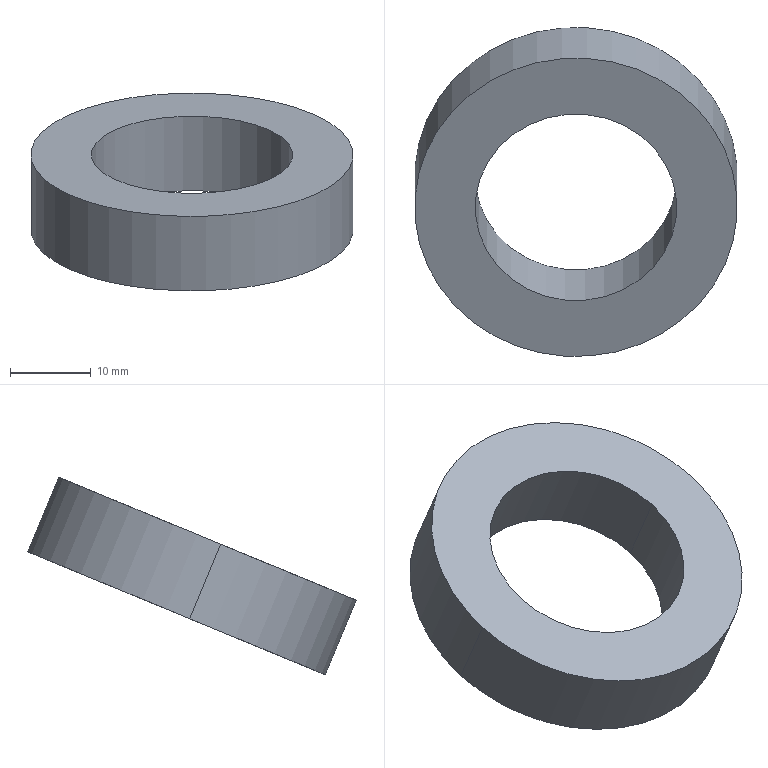Component | SolidWorks | FixedBushing-2 | 1 solid | 6 faces | box 40 x 40.79 x 24.52 mm | volume 7658 mm3 | cylinder 4 | plane 2 | commonest cylinder face diameters 25 x2 40 x2
build123d program:
from build123d import *

# Parameters (mm, degrees)
SKETCH1_R           = 20
SKETCH1_R_2         = 12.5
BOSS_EXTRUDE1_DEPTH = 10


with BuildPart() as part:
    # Sketch1 → Boss-Extrude1 (new body)
    with BuildSketch(Plane.XY):
        Circle(SKETCH1_R)
        Circle(SKETCH1_R_2, mode=Mode.SUBTRACT)
    extrude(amount=BOSS_EXTRUDE1_DEPTH)


solid = part.part

# Placed as in the assembly
solid = solid.moved(Location((-36.329, 8.332, -2.815), (22.448, 0, -44.164)))
STEP:
#1=CARTESIAN_POINT('',(-1.92,0.1377,0.2365));
#2=VERTEX_POINT('',#1);
#3=CARTESIAN_POINT('',(-0.9401,0.2177,0.2696));
#4=VERTEX_POINT('',#3);
#5=CARTESIAN_POINT('',(-1.43,0.1777,0.253));
#6=DIRECTION('',(0.,-0.3818,0.9242));
#7=DIRECTION('',(0.9961,0.0813,0.03359));
#8=AXIS2_PLACEMENT_3D('',#5,#6,#7);
#9=CIRCLE('',#8,0.4921);
#10=EDGE_CURVE('',#2,#4,#9,.T.);
#11=ORIENTED_EDGE('',*,*,#10,.T.);
#12=CARTESIAN_POINT('',(-0.9401,0.368,-0.0943));
#13=VERTEX_POINT('',#12);
#14=CARTESIAN_POINT('',(-0.9401,0.2177,0.2696));
#15=DIRECTION('',(-0.,0.3818,-0.9242));
#16=VECTOR('',#15,39.37);
#17=LINE('',#14,#16);
#18=EDGE_CURVE('',#4,#13,#17,.T.);
#19=ORIENTED_EDGE('',*,*,#18,.T.);
#20=CARTESIAN_POINT('',(-1.92,0.288,-0.1274));
#21=VERTEX_POINT('',#20);
#22=CARTESIAN_POINT('',(-1.43,0.328,-0.1108));
#23=DIRECTION('',(0.,-0.3818,0.9242));
#24=DIRECTION('',(0.9961,0.0813,0.03359));
#25=AXIS2_PLACEMENT_3D('',#22,#23,#24);
#26=CIRCLE('',#25,0.4921);
#27=EDGE_CURVE('',#21,#13,#26,.T.);
#28=ORIENTED_EDGE('',*,*,#27,.F.);
#29=CARTESIAN_POINT('',(-1.92,0.1377,0.2365));
#30=DIRECTION('',(-0.,0.3818,-0.9242));
#31=VECTOR('',#30,39.37);
#32=LINE('',#29,#31);
#33=EDGE_CURVE('',#2,#21,#32,.T.);
#34=ORIENTED_EDGE('',*,*,#33,.F.);
#35=EDGE_LOOP('',(#11,#19,#28,#34));
#36=FACE_OUTER_BOUND('',#35,.T.);
#37=CARTESIAN_POINT('',(-1.43,0.1777,0.253));
#38=DIRECTION('',(-0.,0.3818,-0.9242));
#39=DIRECTION('',(-0.9961,-0.0813,-0.03359));
#40=AXIS2_PLACEMENT_3D('',#37,#38,#39);
#41=CYLINDRICAL_SURFACE('',#40,0.4921);
#42=ADVANCED_FACE('',(#36),#41,.F.);
#43=CARTESIAN_POINT('',(-0.6459,0.2417,0.2795));
#44=VERTEX_POINT('',#43);
#45=CARTESIAN_POINT('',(-2.215,0.1137,0.2266));
#46=VERTEX_POINT('',#45);
#47=CARTESIAN_POINT('',(-1.43,0.1777,0.253));
#48=DIRECTION('',(0.,-0.3818,0.9242));
#49=DIRECTION('',(0.9961,0.0813,0.03359));
#50=AXIS2_PLACEMENT_3D('',#47,#48,#49);
#51=CIRCLE('',#50,0.7874);
#52=EDGE_CURVE('',#44,#46,#51,.T.);
#53=ORIENTED_EDGE('',*,*,#52,.F.);
#54=CARTESIAN_POINT('',(-0.6459,0.392,-0.08439));
#55=VERTEX_POINT('',#54);
#56=CARTESIAN_POINT('',(-0.6459,0.2417,0.2795));
#57=DIRECTION('',(-0.,0.3818,-0.9242));
#58=VECTOR('',#57,39.37);
#59=LINE('',#56,#58);
#60=EDGE_CURVE('',#44,#55,#59,.T.);
#61=ORIENTED_EDGE('',*,*,#60,.T.);
#62=CARTESIAN_POINT('',(-2.215,0.264,-0.1373));
#63=VERTEX_POINT('',#62);
#64=CARTESIAN_POINT('',(-1.43,0.328,-0.1108));
#65=DIRECTION('',(0.,-0.3818,0.9242));
#66=DIRECTION('',(0.9961,0.0813,0.03359));
#67=AXIS2_PLACEMENT_3D('',#64,#65,#66);
#68=CIRCLE('',#67,0.7874);
#69=EDGE_CURVE('',#55,#63,#68,.T.);
#70=ORIENTED_EDGE('',*,*,#69,.T.);
#71=CARTESIAN_POINT('',(-2.215,0.1137,0.2266));
#72=DIRECTION('',(-0.,0.3818,-0.9242));
#73=VECTOR('',#72,39.37);
#74=LINE('',#71,#73);
#75=EDGE_CURVE('',#46,#63,#74,.T.);
#76=ORIENTED_EDGE('',*,*,#75,.F.);
#77=EDGE_LOOP('',(#53,#61,#70,#76));
#78=FACE_OUTER_BOUND('',#77,.T.);
#79=CARTESIAN_POINT('',(-1.43,0.1777,0.253));
#80=DIRECTION('',(-0.,0.3818,-0.9242));
#81=DIRECTION('',(-0.9961,-0.0813,-0.03359));
#82=AXIS2_PLACEMENT_3D('',#79,#80,#81);
#83=CYLINDRICAL_SURFACE('',#82,0.7874);
#84=ADVANCED_FACE('',(#78),#83,.T.);
#85=CARTESIAN_POINT('',(-1.43,0.1777,0.253));
#86=DIRECTION('',(0.,-0.3818,0.9242));
#87=DIRECTION('',(0.9961,0.0813,0.03359));
#88=AXIS2_PLACEMENT_3D('',#85,#86,#87);
#89=CIRCLE('',#88,0.7874);
#90=EDGE_CURVE('',#46,#44,#89,.T.);
#91=ORIENTED_EDGE('',*,*,#90,.T.);
#92=ORIENTED_EDGE('',*,*,#52,.T.);
#93=EDGE_LOOP('',(#91,#92));
#94=FACE_OUTER_BOUND('',#93,.T.);
#95=ORIENTED_EDGE('',*,*,#10,.F.);
#96=CARTESIAN_POINT('',(-1.43,0.1777,0.253));
#97=DIRECTION('',(0.,-0.3818,0.9242));
#98=DIRECTION('',(0.9961,0.0813,0.03359));
#99=AXIS2_PLACEMENT_3D('',#96,#97,#98);
#100=CIRCLE('',#99,0.4921);
#101=EDGE_CURVE('',#4,#2,#100,.T.);
#102=ORIENTED_EDGE('',*,*,#101,.F.);
#103=EDGE_LOOP('',(#95,#102));
#104=FACE_BOUND('',#103,.T.);
#105=CARTESIAN_POINT('',(-1.43,0.1777,0.253));
#106=DIRECTION('',(0.,-0.3818,0.9242));
#107=DIRECTION('',(0.9961,0.0813,0.03359));
#108=AXIS2_PLACEMENT_3D('',#105,#106,#107);
#109=PLANE('',#108);
#110=ADVANCED_FACE('',(#94,#104),#109,.T.);
#111=CARTESIAN_POINT('',(-1.43,0.328,-0.1108));
#112=DIRECTION('',(0.,-0.3818,0.9242));
#113=DIRECTION('',(0.9961,0.0813,0.03359));
#114=AXIS2_PLACEMENT_3D('',#111,#112,#113);
#115=CIRCLE('',#114,0.7874);
#116=EDGE_CURVE('',#63,#55,#115,.T.);
#117=ORIENTED_EDGE('',*,*,#116,.F.);
#118=ORIENTED_EDGE('',*,*,#69,.F.);
#119=EDGE_LOOP('',(#117,#118));
#120=FACE_OUTER_BOUND('',#119,.T.);
#121=ORIENTED_EDGE('',*,*,#27,.T.);
#122=CARTESIAN_POINT('',(-1.43,0.328,-0.1108));
#123=DIRECTION('',(0.,-0.3818,0.9242));
#124=DIRECTION('',(0.9961,0.0813,0.03359));
#125=AXIS2_PLACEMENT_3D('',#122,#123,#124);
#126=CIRCLE('',#125,0.4921);
#127=EDGE_CURVE('',#13,#21,#126,.T.);
#128=ORIENTED_EDGE('',*,*,#127,.T.);
#129=EDGE_LOOP('',(#121,#128));
#130=FACE_BOUND('',#129,.T.);
#131=CARTESIAN_POINT('',(-1.43,0.328,-0.1108));
#132=DIRECTION('',(0.,-0.3818,0.9242));
#133=DIRECTION('',(0.9961,0.0813,0.03359));
#134=AXIS2_PLACEMENT_3D('',#131,#132,#133);
#135=PLANE('',#134);
#136=ADVANCED_FACE('',(#120,#130),#135,.F.);
#137=ORIENTED_EDGE('',*,*,#60,.F.);
#138=ORIENTED_EDGE('',*,*,#90,.F.);
#139=ORIENTED_EDGE('',*,*,#75,.T.);
#140=ORIENTED_EDGE('',*,*,#116,.T.);
#141=EDGE_LOOP('',(#137,#138,#139,#140));
#142=FACE_OUTER_BOUND('',#141,.T.);
#143=CARTESIAN_POINT('',(-1.43,0.1777,0.253));
#144=DIRECTION('',(-0.,0.3818,-0.9242));
#145=DIRECTION('',(-0.9961,-0.0813,-0.03359));
#146=AXIS2_PLACEMENT_3D('',#143,#144,#145);
#147=CYLINDRICAL_SURFACE('',#146,0.7874);
#148=ADVANCED_FACE('',(#142),#147,.T.);
#149=ORIENTED_EDGE('',*,*,#18,.F.);
#150=ORIENTED_EDGE('',*,*,#101,.T.);
#151=ORIENTED_EDGE('',*,*,#33,.T.);
#152=ORIENTED_EDGE('',*,*,#127,.F.);
#153=EDGE_LOOP('',(#149,#150,#151,#152));
#154=FACE_OUTER_BOUND('',#153,.T.);
#155=CARTESIAN_POINT('',(-1.43,0.1777,0.253));
#156=DIRECTION('',(-0.,0.3818,-0.9242));
#157=DIRECTION('',(-0.9961,-0.0813,-0.03359));
#158=AXIS2_PLACEMENT_3D('',#155,#156,#157);
#159=CYLINDRICAL_SURFACE('',#158,0.4921);
#160=ADVANCED_FACE('',(#154),#159,.F.);
#161=CLOSED_SHELL('',(#42,#84,#110,#136,#148,#160));
#162=MANIFOLD_SOLID_BREP('',#161);
#163=CARTESIAN_POINT('',(0.,0.,0.));
#164=DIRECTION('',(0.,0.,1.));
#165=DIRECTION('',(1.,0.,0.));
#166=AXIS2_PLACEMENT_3D('',#163,#164,#165);
#167=(LENGTH_UNIT()NAMED_UNIT(*)SI_UNIT($,.METRE.));
#168=LENGTH_MEASURE_WITH_UNIT(LENGTH_MEASURE(0.0254),#167);
#169=DIMENSIONAL_EXPONENTS(1.,0.,0.,0.,0.,0.,0.);
#170=(CONVERSION_BASED_UNIT('',#168)LENGTH_UNIT()NAMED_UNIT(#169));
#171=UNCERTAINTY_MEASURE_WITH_UNIT(LENGTH_MEASURE(0.00001),#170,'','');
#172=(NAMED_UNIT(*)PLANE_ANGLE_UNIT()SI_UNIT($,.RADIAN.));
#173=(NAMED_UNIT(*)SI_UNIT($,.STERADIAN.)SOLID_ANGLE_UNIT());
#174=(GEOMETRIC_REPRESENTATION_CONTEXT(3)GLOBAL_UNCERTAINTY_ASSIGNED_CONTEXT((#171))GLOBAL_UNIT_ASSIGNED_CONTEXT((#170,#172,#173))REPRESENTATION_CONTEXT('',''));
#175=ADVANCED_BREP_SHAPE_REPRESENTATION('',(#162,#166),#174);
#176=COLOUR_RGB('',0.7922,0.8196,0.9333);
#177=FILL_AREA_STYLE_COLOUR('',#176);
#178=FILL_AREA_STYLE('',(#177));
#179=SURFACE_STYLE_FILL_AREA(#178);
#180=SURFACE_SIDE_STYLE('',(#179));
#181=SURFACE_STYLE_USAGE(.BOTH.,#180);
#182=PRESENTATION_STYLE_ASSIGNMENT((#181));
#183=STYLED_ITEM('',(#182),#162);
#184=PRESENTATION_LAYER_ASSIGNMENT('','',(#183));
#185=(LENGTH_UNIT()NAMED_UNIT(*)SI_UNIT($,.METRE.));
#186=LENGTH_MEASURE_WITH_UNIT(LENGTH_MEASURE(0.0254),#185);
#187=DIMENSIONAL_EXPONENTS(1.,0.,0.,0.,0.,0.,0.);
#188=(CONVERSION_BASED_UNIT('',#186)LENGTH_UNIT()NAMED_UNIT(#187));
#189=UNCERTAINTY_MEASURE_WITH_UNIT(LENGTH_MEASURE(0.00001),#188,'','');
#190=(NAMED_UNIT(*)PLANE_ANGLE_UNIT()SI_UNIT($,.RADIAN.));
#191=(NAMED_UNIT(*)SI_UNIT($,.STERADIAN.)SOLID_ANGLE_UNIT());
#192=(GEOMETRIC_REPRESENTATION_CONTEXT(3)GLOBAL_UNCERTAINTY_ASSIGNED_CONTEXT((#189))GLOBAL_UNIT_ASSIGNED_CONTEXT((#188,#190,#191))REPRESENTATION_CONTEXT('',''));
#193=MECHANICAL_DESIGN_GEOMETRIC_PRESENTATION_REPRESENTATION('',(#183),#192);